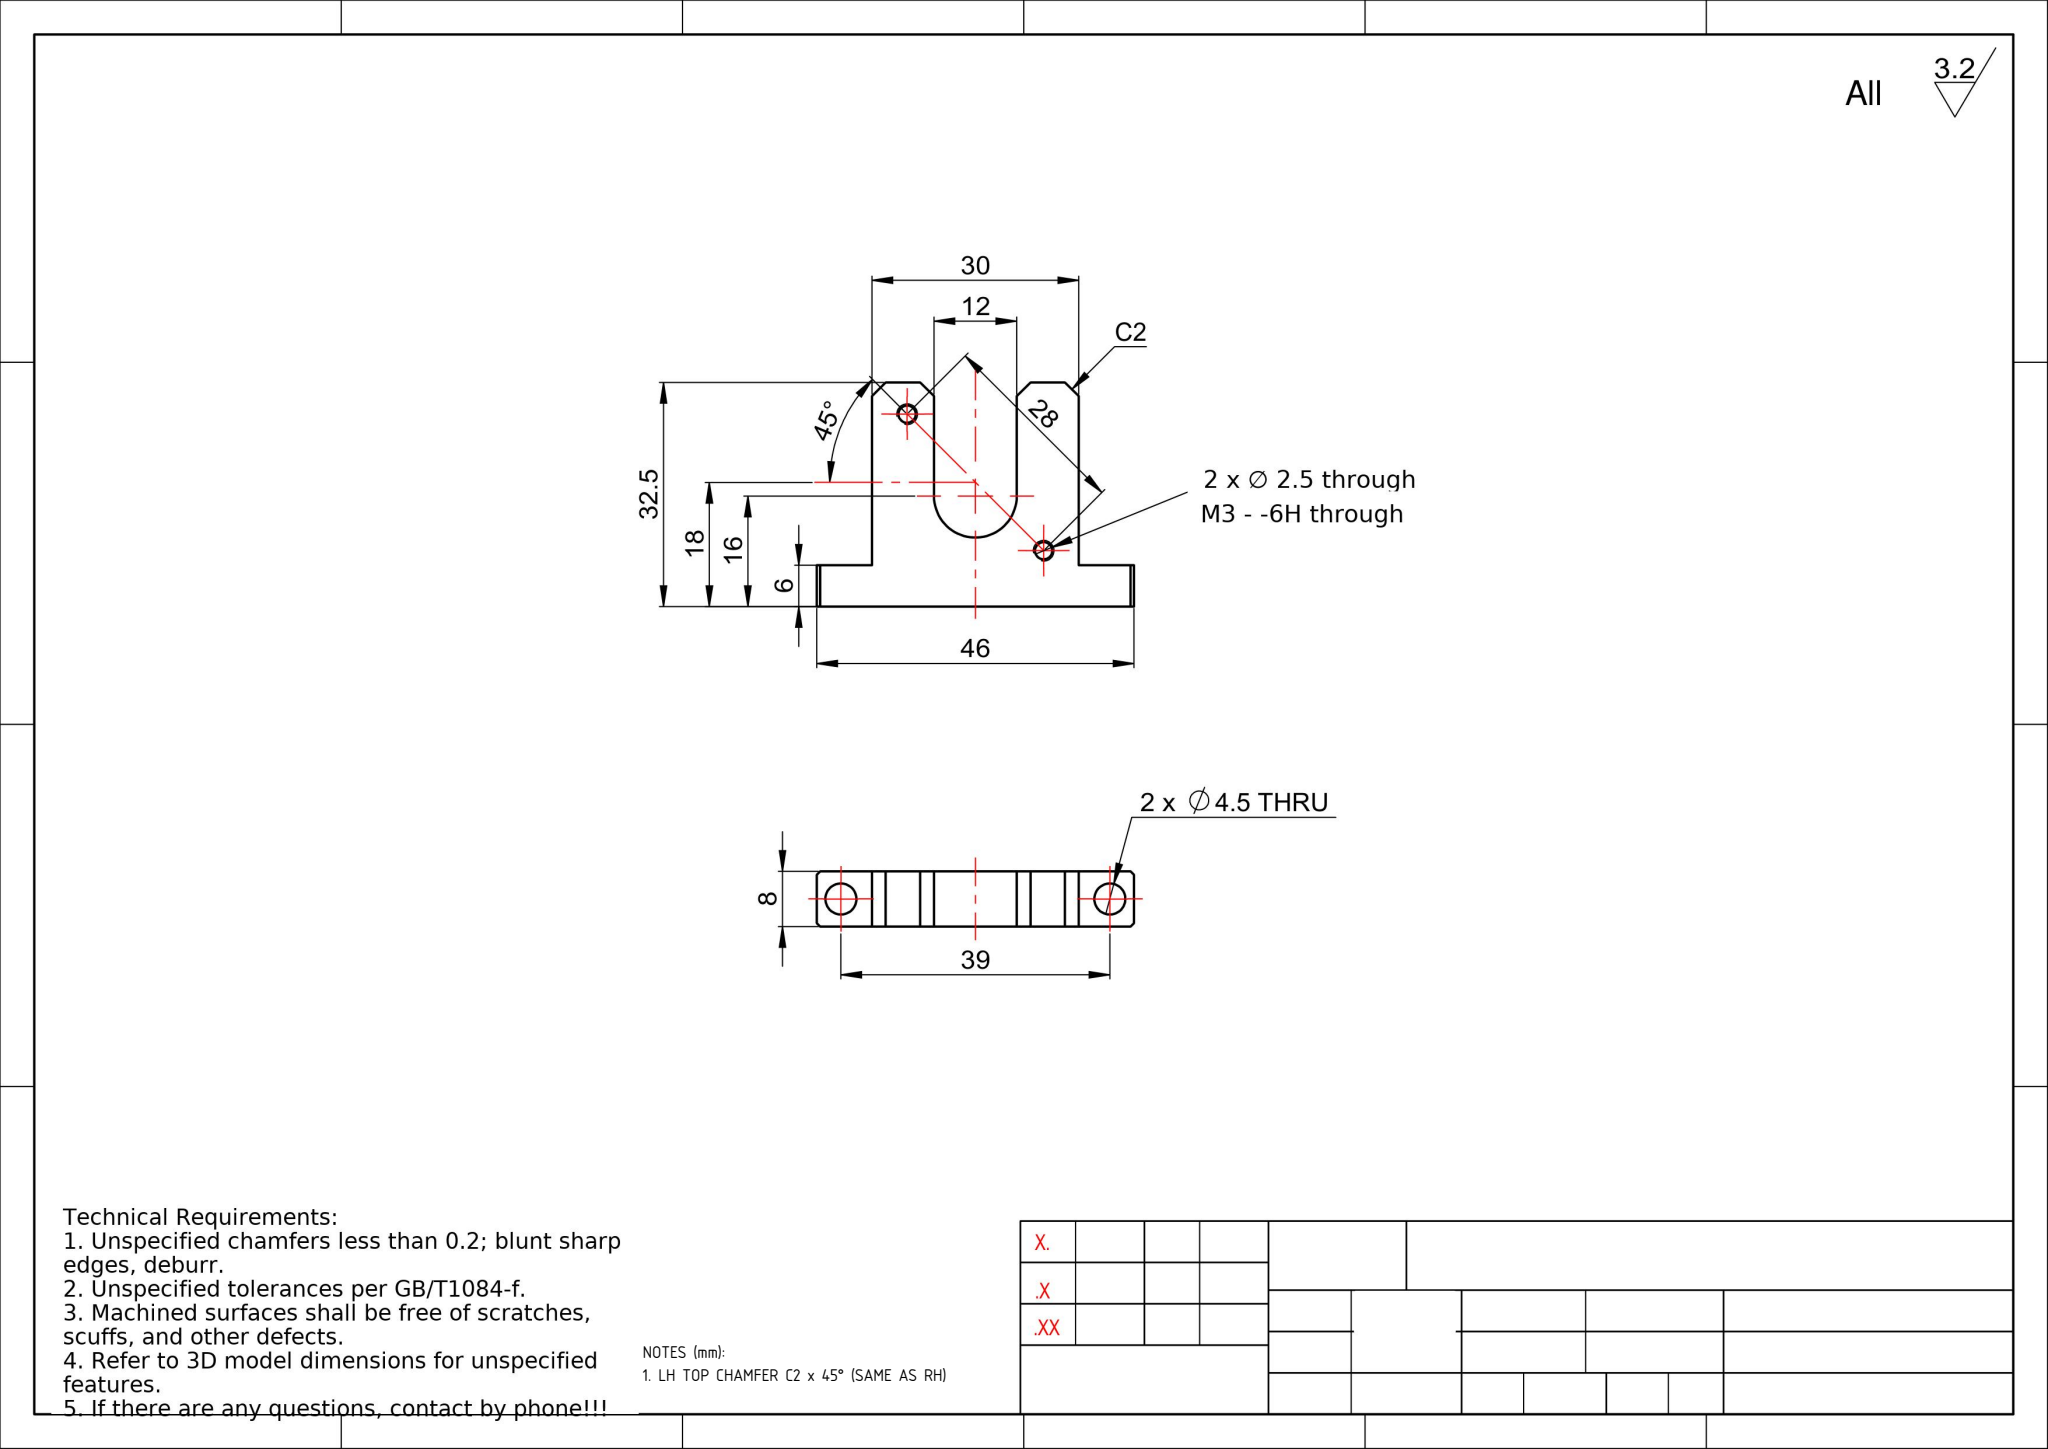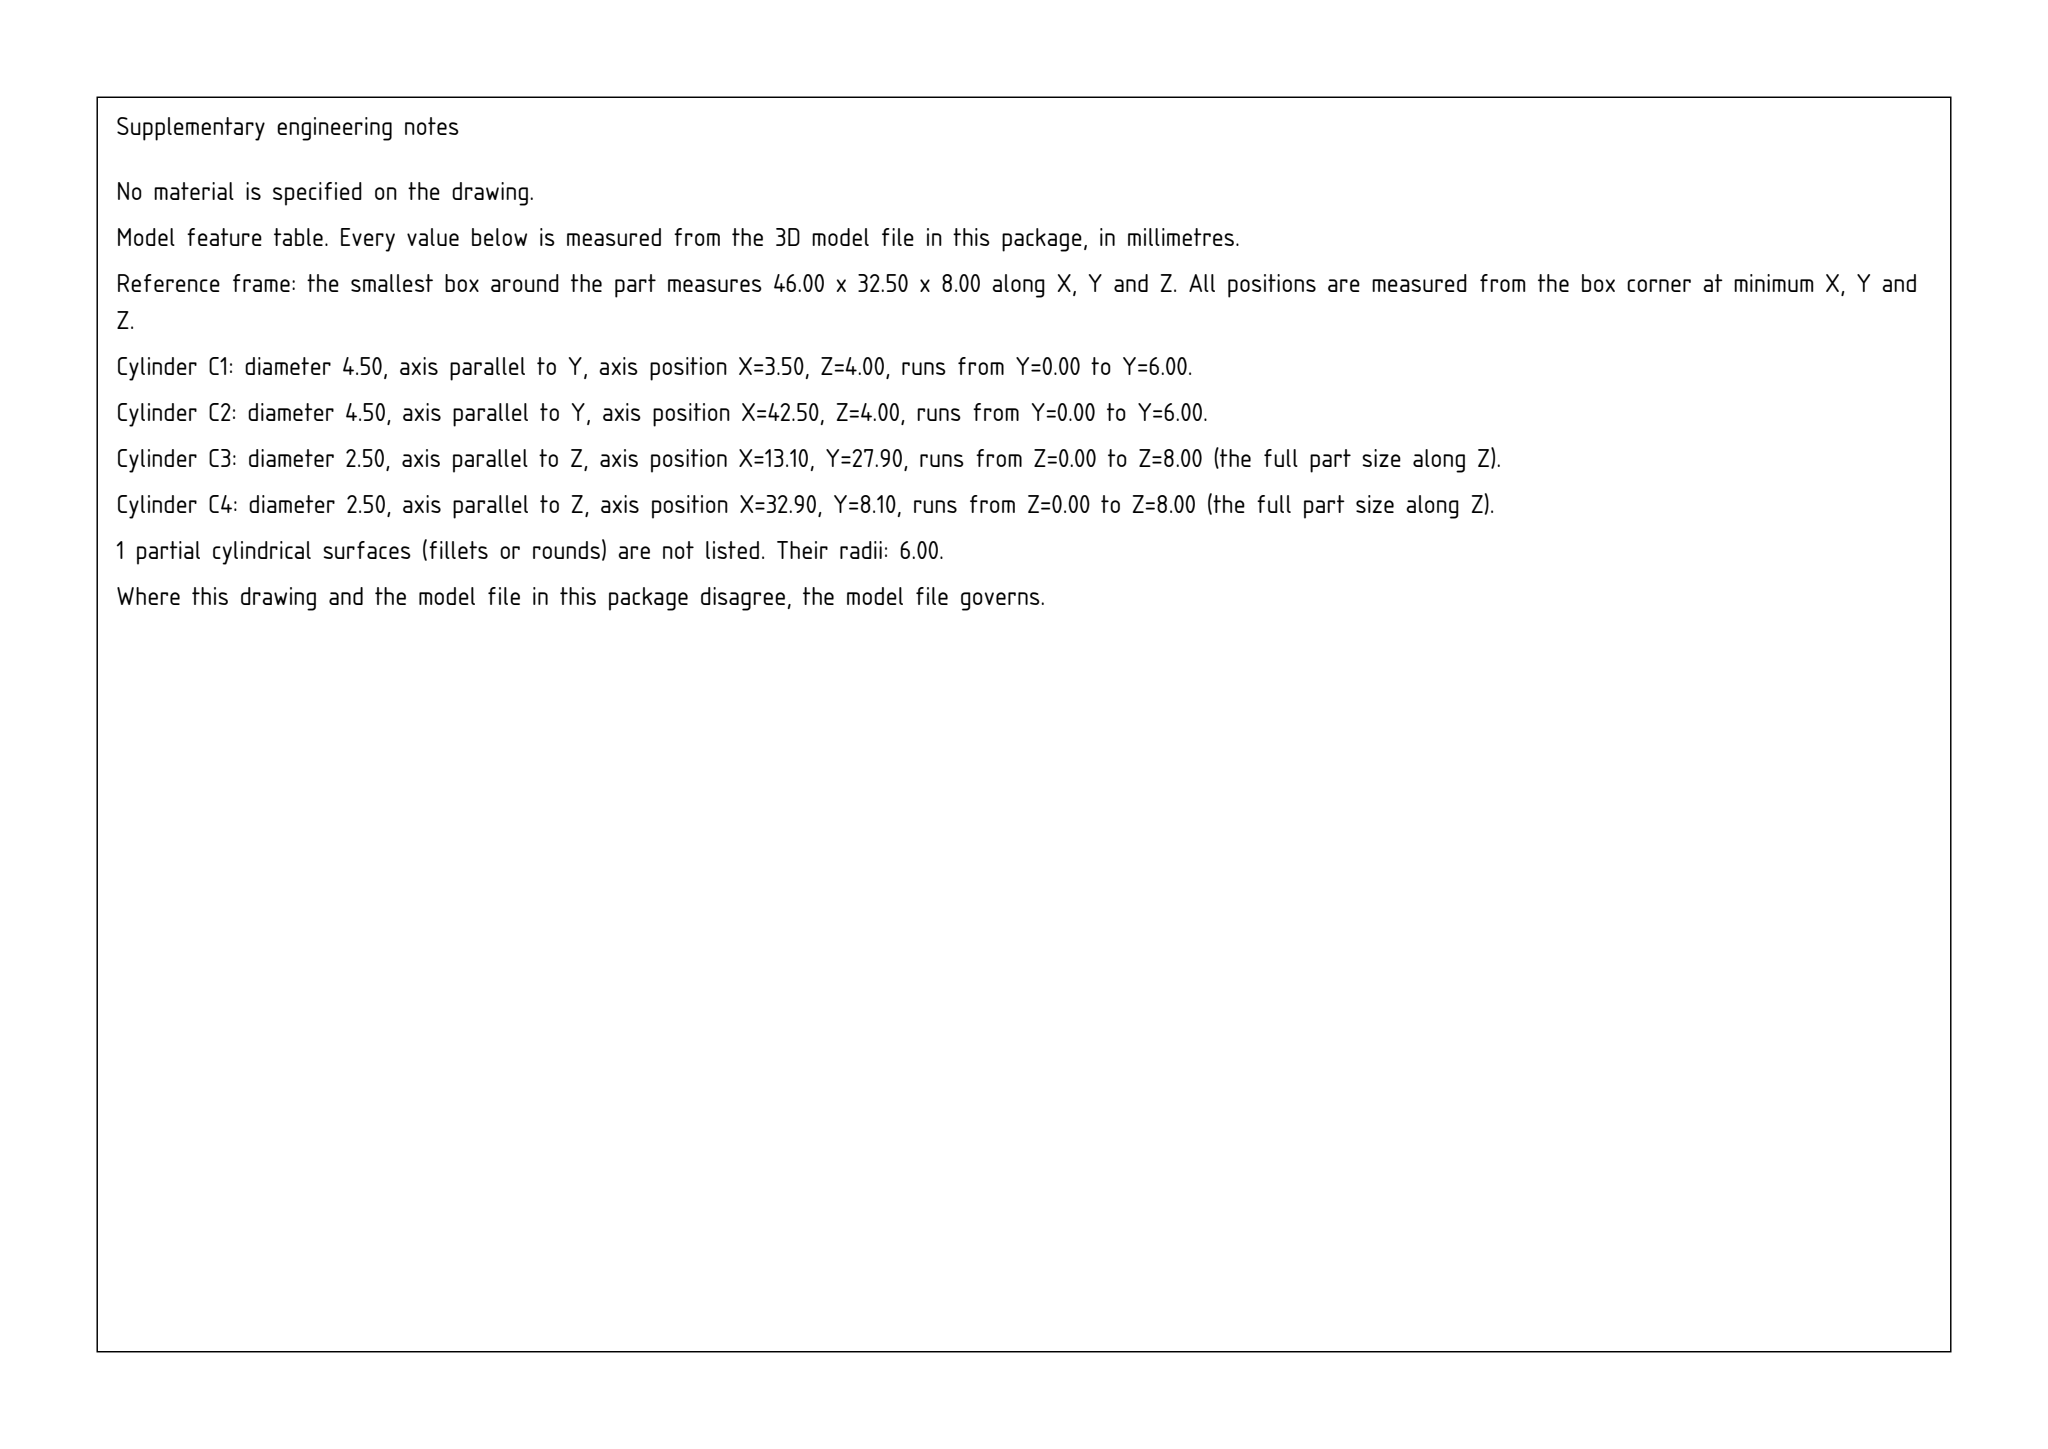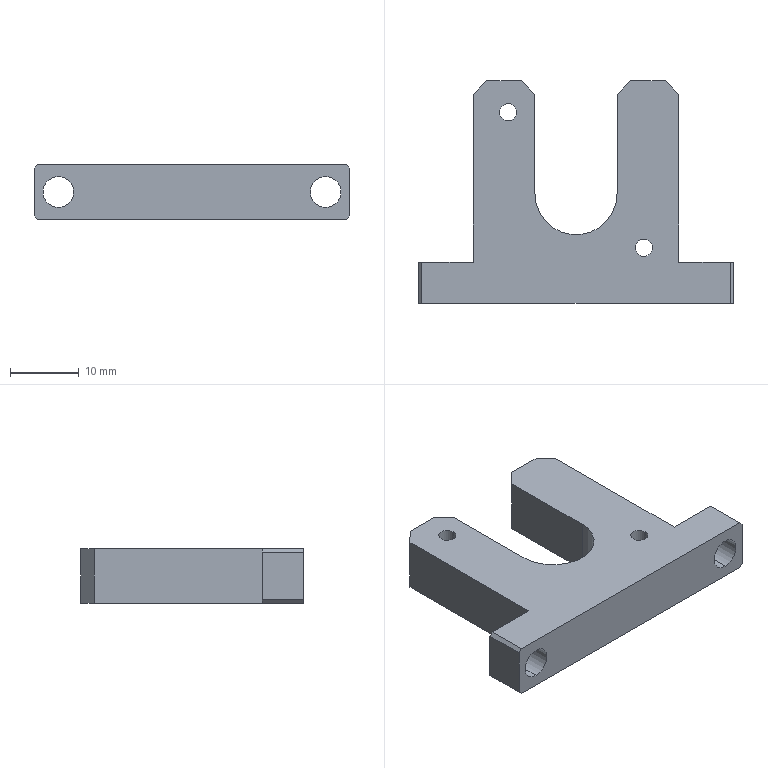Part | SolidWorks | mm | 1 solid | 30 faces | box 46 x 32.5 x 8 mm | volume 6195 mm3 | plane 21 | cylinder 9 | commonest cylinder face diameters 4.5 x4 2.5 x4 12 x1
Drawing notes:
LH TOP CHAMFER C2 x 45° (SAME AS RH) | from the solid: Upright top face y=32.5 spans x=8..38 (30 wide); symmetric top corner breaks, RH chamfer C2 at x=38 corner, LH mirror at x=8 corner
build123d program:
from build123d import *

# Parameters (mm, degrees)
SKETCH1_W                  = 30
SKETCH1_H                  = 32.5
BOSS_EXTRUDE1_DEPTH        = 4
CHAMFER1_SIZE              = 2
CUT_EXTRUDE2_DEPTH         = 24.517
CHAMFER2_SIZE              = 2
M3_TAPPED_HOLE1_D          = 2.5
SKETCH7_W                  = 8
SKETCH7_H                  = 6
BOSS_EXTRUDE2_DEPTH        = 8
F_4_5_4_5_DIAMETER_HOLE1_D = 4.5
CHAMFER3_SIZE              = 0.5


with BuildPart() as part:
    # Sketch1 → Boss-Extrude1 (new, symmetric)
    with BuildSketch(Plane.XY):
        Rectangle(SKETCH1_W, SKETCH1_H)
    extrude(amount=BOSS_EXTRUDE1_DEPTH, both=True)

    # Chamfer1
    chamfer1_edges = [part.edges().sort_by_distance(p)[0] for p in [
        (-15, 16.25, 0),
        (15, 16.25, 0),
    ]]
    chamfer(chamfer1_edges, length=CHAMFER1_SIZE)

    # Sketch4 → Cut-Extrude2 (cut, through all)
    with BuildSketch(Plane.XY.offset(4)):
        with BuildLine():
            Line((-6, -0.25), (-6, 16.25))
            Line((-6, 16.25), (6, 16.25))
            Line((6, 16.25), (6, -0.25))
            ThreePointArc((6, -0.25), (0, -6.25), (-6, -0.25))
        make_face()
    extrude(amount=-CUT_EXTRUDE2_DEPTH, mode=Mode.SUBTRACT)

    # Chamfer2
    chamfer2_edges = [part.edges().sort_by_distance(p)[0] for p in [
        (-6, 16.25, 0),
        (6, 16.25, 0),
    ]]
    chamfer(chamfer2_edges, length=CHAMFER2_SIZE)

    # M3 Tapped Hole1 (through all)
    with Locations(Plane.XY.offset(4)):
        with Locations((-9.899, 11.649), (9.899, -8.15)):
            Hole(M3_TAPPED_HOLE1_D / 2)

    # Sketch7 → Boss-Extrude2 (add)
    with BuildSketch(Plane(origin=(0, 0, -4), x_dir=(-1, 0, 0), z_dir=(0, 0, -1))):
        with Locations((-19, -13.25)):
            Rectangle(SKETCH7_W, SKETCH7_H)
        with Locations((19, -13.25)):
            Rectangle(SKETCH7_W, SKETCH7_H)
    extrude(amount=-BOSS_EXTRUDE2_DEPTH)

    # 4.5 _4.5_ Diameter Hole1 (through all)
    with Locations(Plane(origin=(0, -10.25, 0), x_dir=(1, 0, 0), z_dir=(0, 1, 0))):
        with Locations((19.5, 0), (-19.5, 0)):
            Hole(F_4_5_4_5_DIAMETER_HOLE1_D / 2)

    # Chamfer3
    chamfer3_edges = [part.edges().sort_by_distance(p)[0] for p in [
        (23, -13.25, -4),
        (23, -13.25, 4),
        (-23, -13.25, -4),
        (-23, -13.25, 4),
    ]]
    chamfer(chamfer3_edges, length=CHAMFER3_SIZE)


solid = part.part